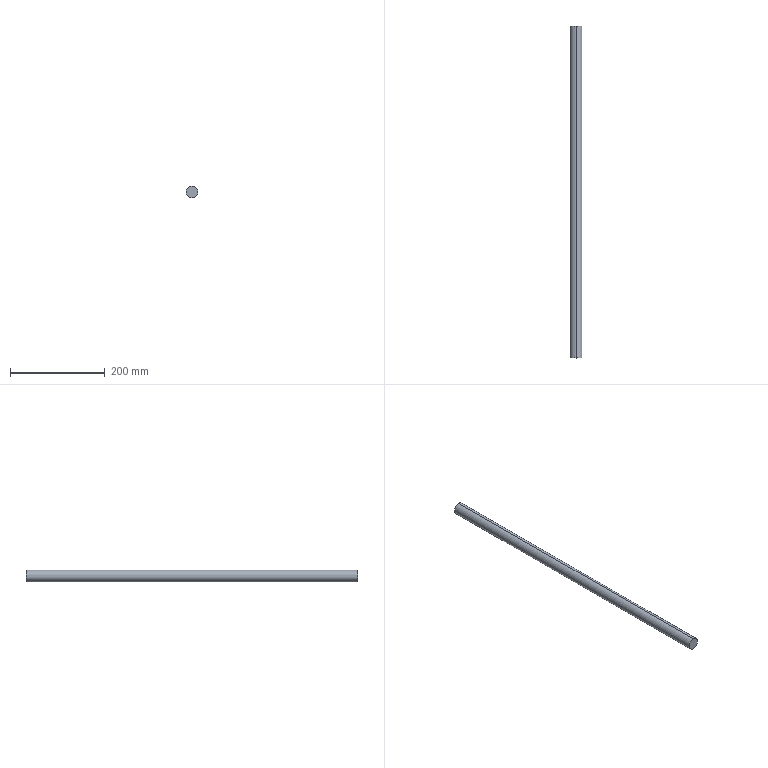Component | SolidWorks | GuideRod-331-1 | 1 solid | 4 faces | box 25 x 700 x 25 mm | volume 343612 mm3 | cylinder 2 | plane 2 | commonest cylinder face diameters 25 x2
build123d program:
from build123d import *

# Parameters (mm, degrees)
SKETCH1_R           = 12.5
BOSS_EXTRUDE1_DEPTH = 700


with BuildPart() as part:
    # Sketch1 → Boss-Extrude1 (new body)
    with BuildSketch(Plane(origin=(0, 0, 0), x_dir=(1, 0, 0), z_dir=(0, 1, 0))):
        with Locations(Location((0, 0, 0), (0, 0, 270))):
            Circle(SKETCH1_R)
    extrude(amount=BOSS_EXTRUDE1_DEPTH)


solid = part.part

# Placed as in the assembly
solid = solid.moved(Location((-181.681, 605.897, 683.723), (0, 0, 0)))
STEP:
#1=CARTESIAN_POINT('',(-7.153,51.413,27.41));
#2=VERTEX_POINT('',#1);
#3=CARTESIAN_POINT('',(-7.153,51.413,26.426));
#4=VERTEX_POINT('',#3);
#5=CARTESIAN_POINT('',(-7.153,51.413,26.918));
#6=DIRECTION('',(0.,1.,0.));
#7=DIRECTION('',(0.,0.,1.));
#8=AXIS2_PLACEMENT_3D('',#5,#6,#7);
#9=CIRCLE('',#8,0.4921);
#10=EDGE_CURVE('',#2,#4,#9,.T.);
#11=ORIENTED_EDGE('',*,*,#10,.F.);
#12=CARTESIAN_POINT('',(-7.153,23.854,27.41));
#13=VERTEX_POINT('',#12);
#14=CARTESIAN_POINT('',(-7.153,51.413,27.41));
#15=DIRECTION('',(0.,-1.,0.));
#16=VECTOR('',#15,39.37);
#17=LINE('',#14,#16);
#18=EDGE_CURVE('',#2,#13,#17,.T.);
#19=ORIENTED_EDGE('',*,*,#18,.T.);
#20=CARTESIAN_POINT('',(-7.153,23.854,26.426));
#21=VERTEX_POINT('',#20);
#22=CARTESIAN_POINT('',(-7.153,23.854,26.918));
#23=DIRECTION('',(0.,1.,0.));
#24=DIRECTION('',(0.,0.,1.));
#25=AXIS2_PLACEMENT_3D('',#22,#23,#24);
#26=CIRCLE('',#25,0.4921);
#27=EDGE_CURVE('',#13,#21,#26,.T.);
#28=ORIENTED_EDGE('',*,*,#27,.T.);
#29=CARTESIAN_POINT('',(-7.153,51.413,26.426));
#30=DIRECTION('',(0.,-1.,0.));
#31=VECTOR('',#30,39.37);
#32=LINE('',#29,#31);
#33=EDGE_CURVE('',#4,#21,#32,.T.);
#34=ORIENTED_EDGE('',*,*,#33,.F.);
#35=EDGE_LOOP('',(#11,#19,#28,#34));
#36=FACE_OUTER_BOUND('',#35,.T.);
#37=CARTESIAN_POINT('',(-7.153,51.413,26.918));
#38=DIRECTION('',(0.,-1.,0.));
#39=DIRECTION('',(0.,0.,-1.));
#40=AXIS2_PLACEMENT_3D('',#37,#38,#39);
#41=CYLINDRICAL_SURFACE('',#40,0.4921);
#42=ADVANCED_FACE('',(#36),#41,.T.);
#43=ORIENTED_EDGE('',*,*,#18,.F.);
#44=CARTESIAN_POINT('',(-7.153,51.413,26.918));
#45=DIRECTION('',(0.,1.,0.));
#46=DIRECTION('',(0.,0.,1.));
#47=AXIS2_PLACEMENT_3D('',#44,#45,#46);
#48=CIRCLE('',#47,0.4921);
#49=EDGE_CURVE('',#4,#2,#48,.T.);
#50=ORIENTED_EDGE('',*,*,#49,.F.);
#51=ORIENTED_EDGE('',*,*,#33,.T.);
#52=CARTESIAN_POINT('',(-7.153,23.854,26.918));
#53=DIRECTION('',(0.,1.,0.));
#54=DIRECTION('',(0.,0.,1.));
#55=AXIS2_PLACEMENT_3D('',#52,#53,#54);
#56=CIRCLE('',#55,0.4921);
#57=EDGE_CURVE('',#21,#13,#56,.T.);
#58=ORIENTED_EDGE('',*,*,#57,.T.);
#59=EDGE_LOOP('',(#43,#50,#51,#58));
#60=FACE_OUTER_BOUND('',#59,.T.);
#61=CARTESIAN_POINT('',(-7.153,51.413,26.918));
#62=DIRECTION('',(0.,-1.,0.));
#63=DIRECTION('',(0.,0.,-1.));
#64=AXIS2_PLACEMENT_3D('',#61,#62,#63);
#65=CYLINDRICAL_SURFACE('',#64,0.4921);
#66=ADVANCED_FACE('',(#60),#65,.T.);
#67=ORIENTED_EDGE('',*,*,#49,.T.);
#68=ORIENTED_EDGE('',*,*,#10,.T.);
#69=EDGE_LOOP('',(#67,#68));
#70=FACE_OUTER_BOUND('',#69,.T.);
#71=CARTESIAN_POINT('',(-7.153,51.413,26.918));
#72=DIRECTION('',(0.,1.,0.));
#73=DIRECTION('',(0.,0.,1.));
#74=AXIS2_PLACEMENT_3D('',#71,#72,#73);
#75=PLANE('',#74);
#76=ADVANCED_FACE('',(#70),#75,.T.);
#77=ORIENTED_EDGE('',*,*,#57,.F.);
#78=ORIENTED_EDGE('',*,*,#27,.F.);
#79=EDGE_LOOP('',(#77,#78));
#80=FACE_OUTER_BOUND('',#79,.T.);
#81=CARTESIAN_POINT('',(-7.153,23.854,26.918));
#82=DIRECTION('',(0.,1.,0.));
#83=DIRECTION('',(0.,0.,1.));
#84=AXIS2_PLACEMENT_3D('',#81,#82,#83);
#85=PLANE('',#84);
#86=ADVANCED_FACE('',(#80),#85,.F.);
#87=CLOSED_SHELL('',(#42,#66,#76,#86));
#88=MANIFOLD_SOLID_BREP('',#87);
#89=CARTESIAN_POINT('',(0.,0.,0.));
#90=DIRECTION('',(0.,0.,1.));
#91=DIRECTION('',(1.,0.,0.));
#92=AXIS2_PLACEMENT_3D('',#89,#90,#91);
#93=(LENGTH_UNIT()NAMED_UNIT(*)SI_UNIT($,.METRE.));
#94=LENGTH_MEASURE_WITH_UNIT(LENGTH_MEASURE(0.0254),#93);
#95=DIMENSIONAL_EXPONENTS(1.,0.,0.,0.,0.,0.,0.);
#96=(CONVERSION_BASED_UNIT('',#94)LENGTH_UNIT()NAMED_UNIT(#95));
#97=UNCERTAINTY_MEASURE_WITH_UNIT(LENGTH_MEASURE(0.00001),#96,'','');
#98=(NAMED_UNIT(*)PLANE_ANGLE_UNIT()SI_UNIT($,.RADIAN.));
#99=(NAMED_UNIT(*)SI_UNIT($,.STERADIAN.)SOLID_ANGLE_UNIT());
#100=(GEOMETRIC_REPRESENTATION_CONTEXT(3)GLOBAL_UNCERTAINTY_ASSIGNED_CONTEXT((#97))GLOBAL_UNIT_ASSIGNED_CONTEXT((#96,#98,#99))REPRESENTATION_CONTEXT('',''));
#101=ADVANCED_BREP_SHAPE_REPRESENTATION('',(#88,#92),#100);
#102=COLOUR_RGB('',0.7922,0.8196,0.9333);
#103=FILL_AREA_STYLE_COLOUR('',#102);
#104=FILL_AREA_STYLE('',(#103));
#105=SURFACE_STYLE_FILL_AREA(#104);
#106=SURFACE_SIDE_STYLE('',(#105));
#107=SURFACE_STYLE_USAGE(.BOTH.,#106);
#108=PRESENTATION_STYLE_ASSIGNMENT((#107));
#109=STYLED_ITEM('',(#108),#88);
#110=PRESENTATION_LAYER_ASSIGNMENT('','',(#109));
#111=(LENGTH_UNIT()NAMED_UNIT(*)SI_UNIT($,.METRE.));
#112=LENGTH_MEASURE_WITH_UNIT(LENGTH_MEASURE(0.0254),#111);
#113=DIMENSIONAL_EXPONENTS(1.,0.,0.,0.,0.,0.,0.);
#114=(CONVERSION_BASED_UNIT('',#112)LENGTH_UNIT()NAMED_UNIT(#113));
#115=UNCERTAINTY_MEASURE_WITH_UNIT(LENGTH_MEASURE(0.00001),#114,'','');
#116=(NAMED_UNIT(*)PLANE_ANGLE_UNIT()SI_UNIT($,.RADIAN.));
#117=(NAMED_UNIT(*)SI_UNIT($,.STERADIAN.)SOLID_ANGLE_UNIT());
#118=(GEOMETRIC_REPRESENTATION_CONTEXT(3)GLOBAL_UNCERTAINTY_ASSIGNED_CONTEXT((#115))GLOBAL_UNIT_ASSIGNED_CONTEXT((#114,#116,#117))REPRESENTATION_CONTEXT('',''));
#119=MECHANICAL_DESIGN_GEOMETRIC_PRESENTATION_REPRESENTATION('',(#109),#118);